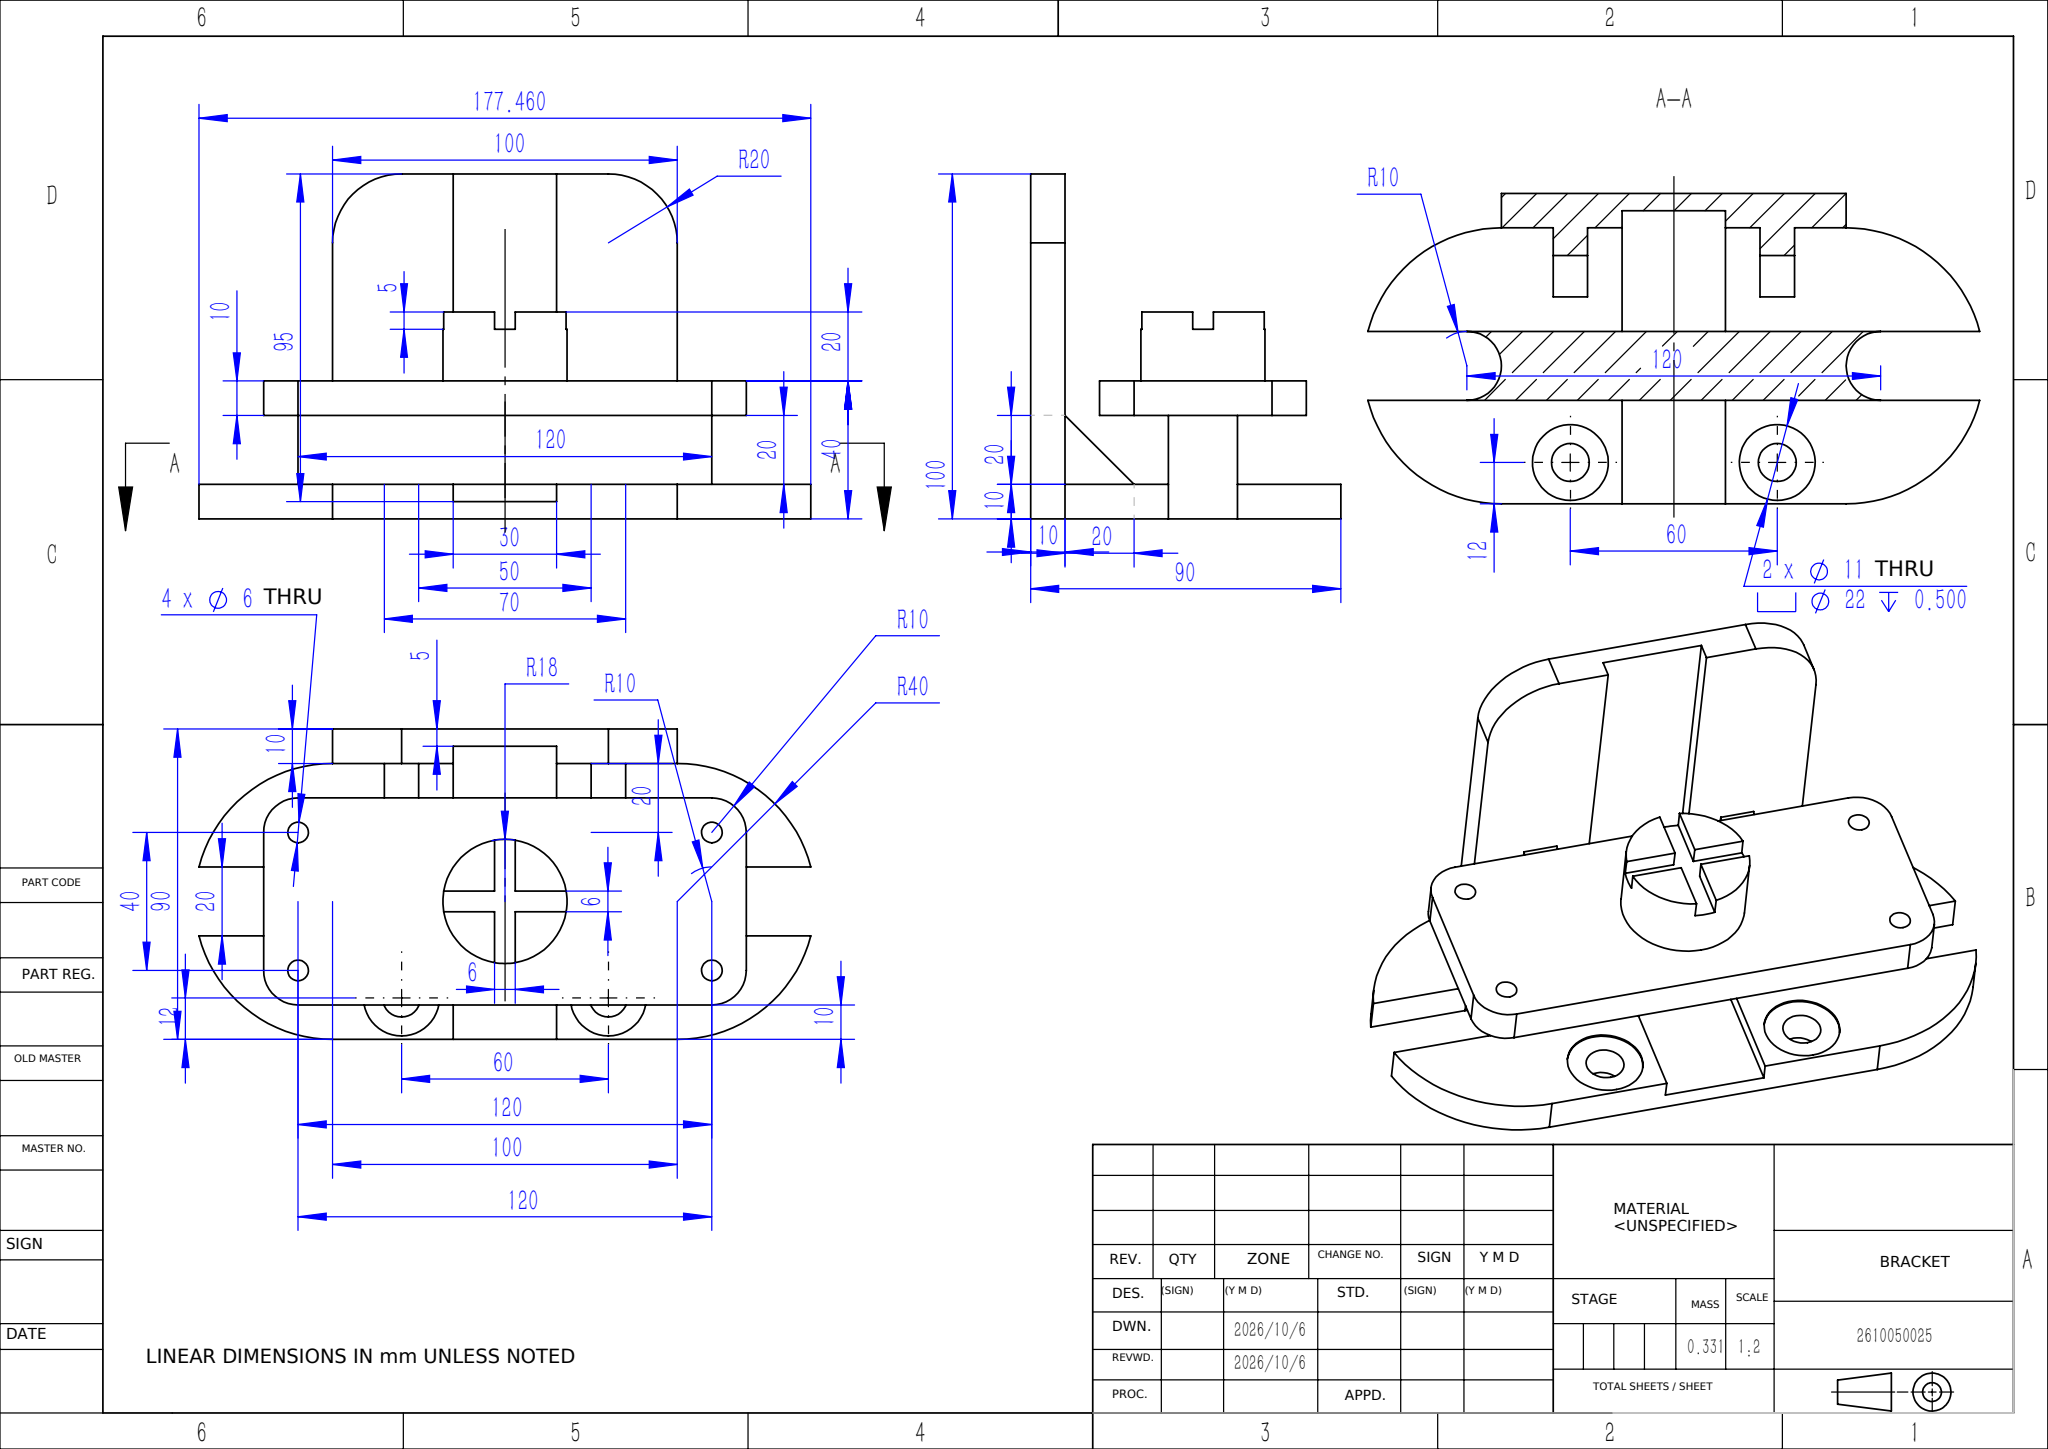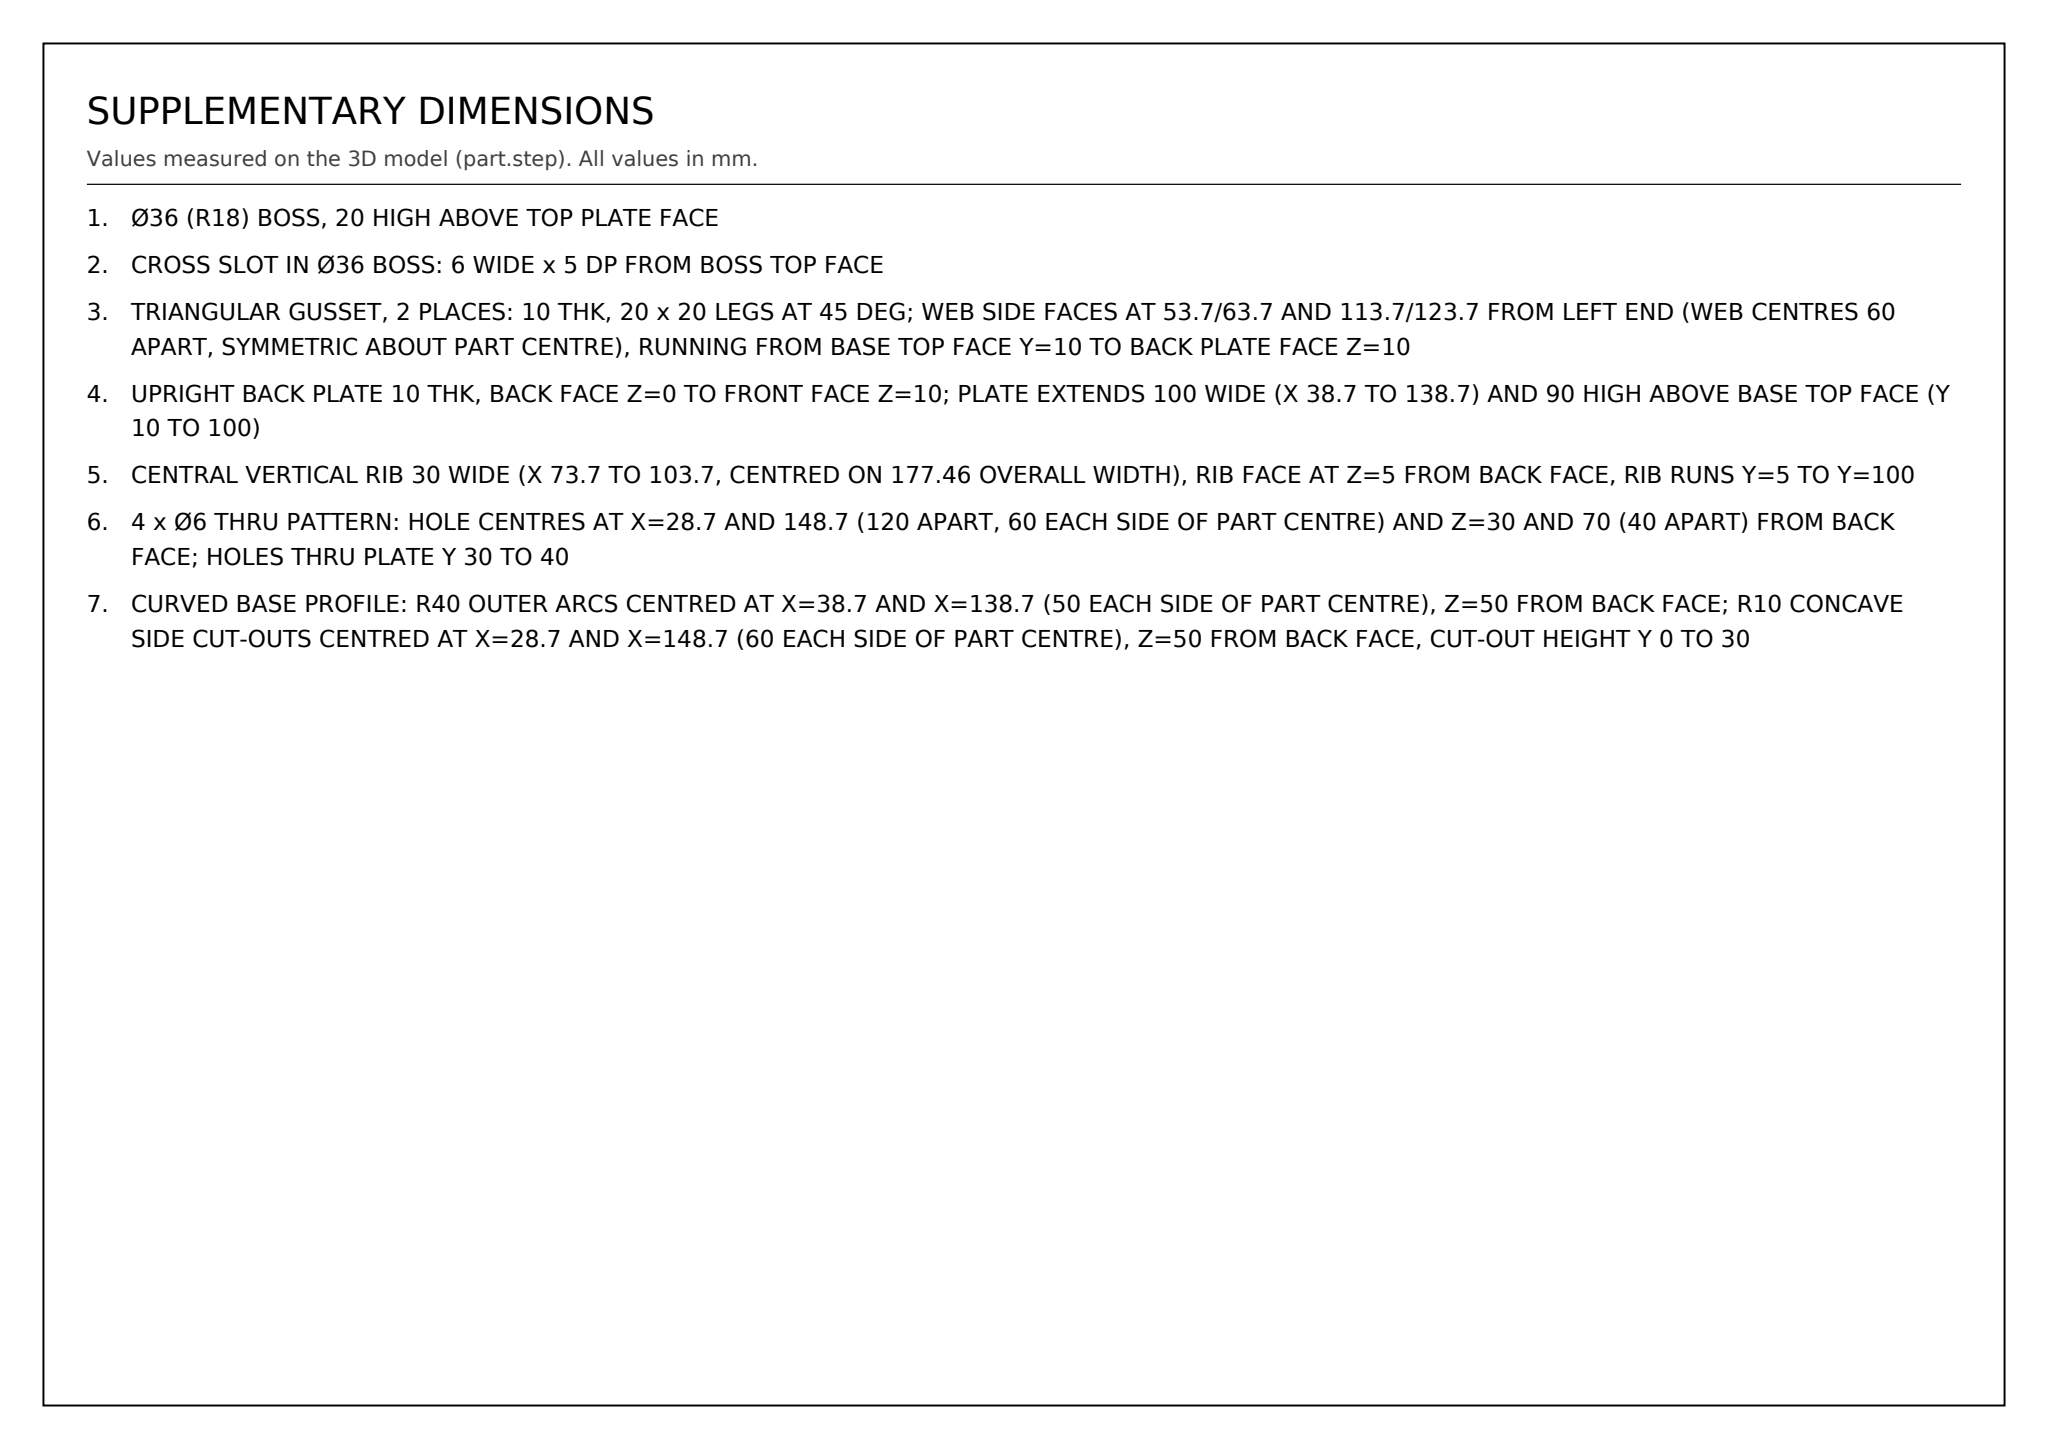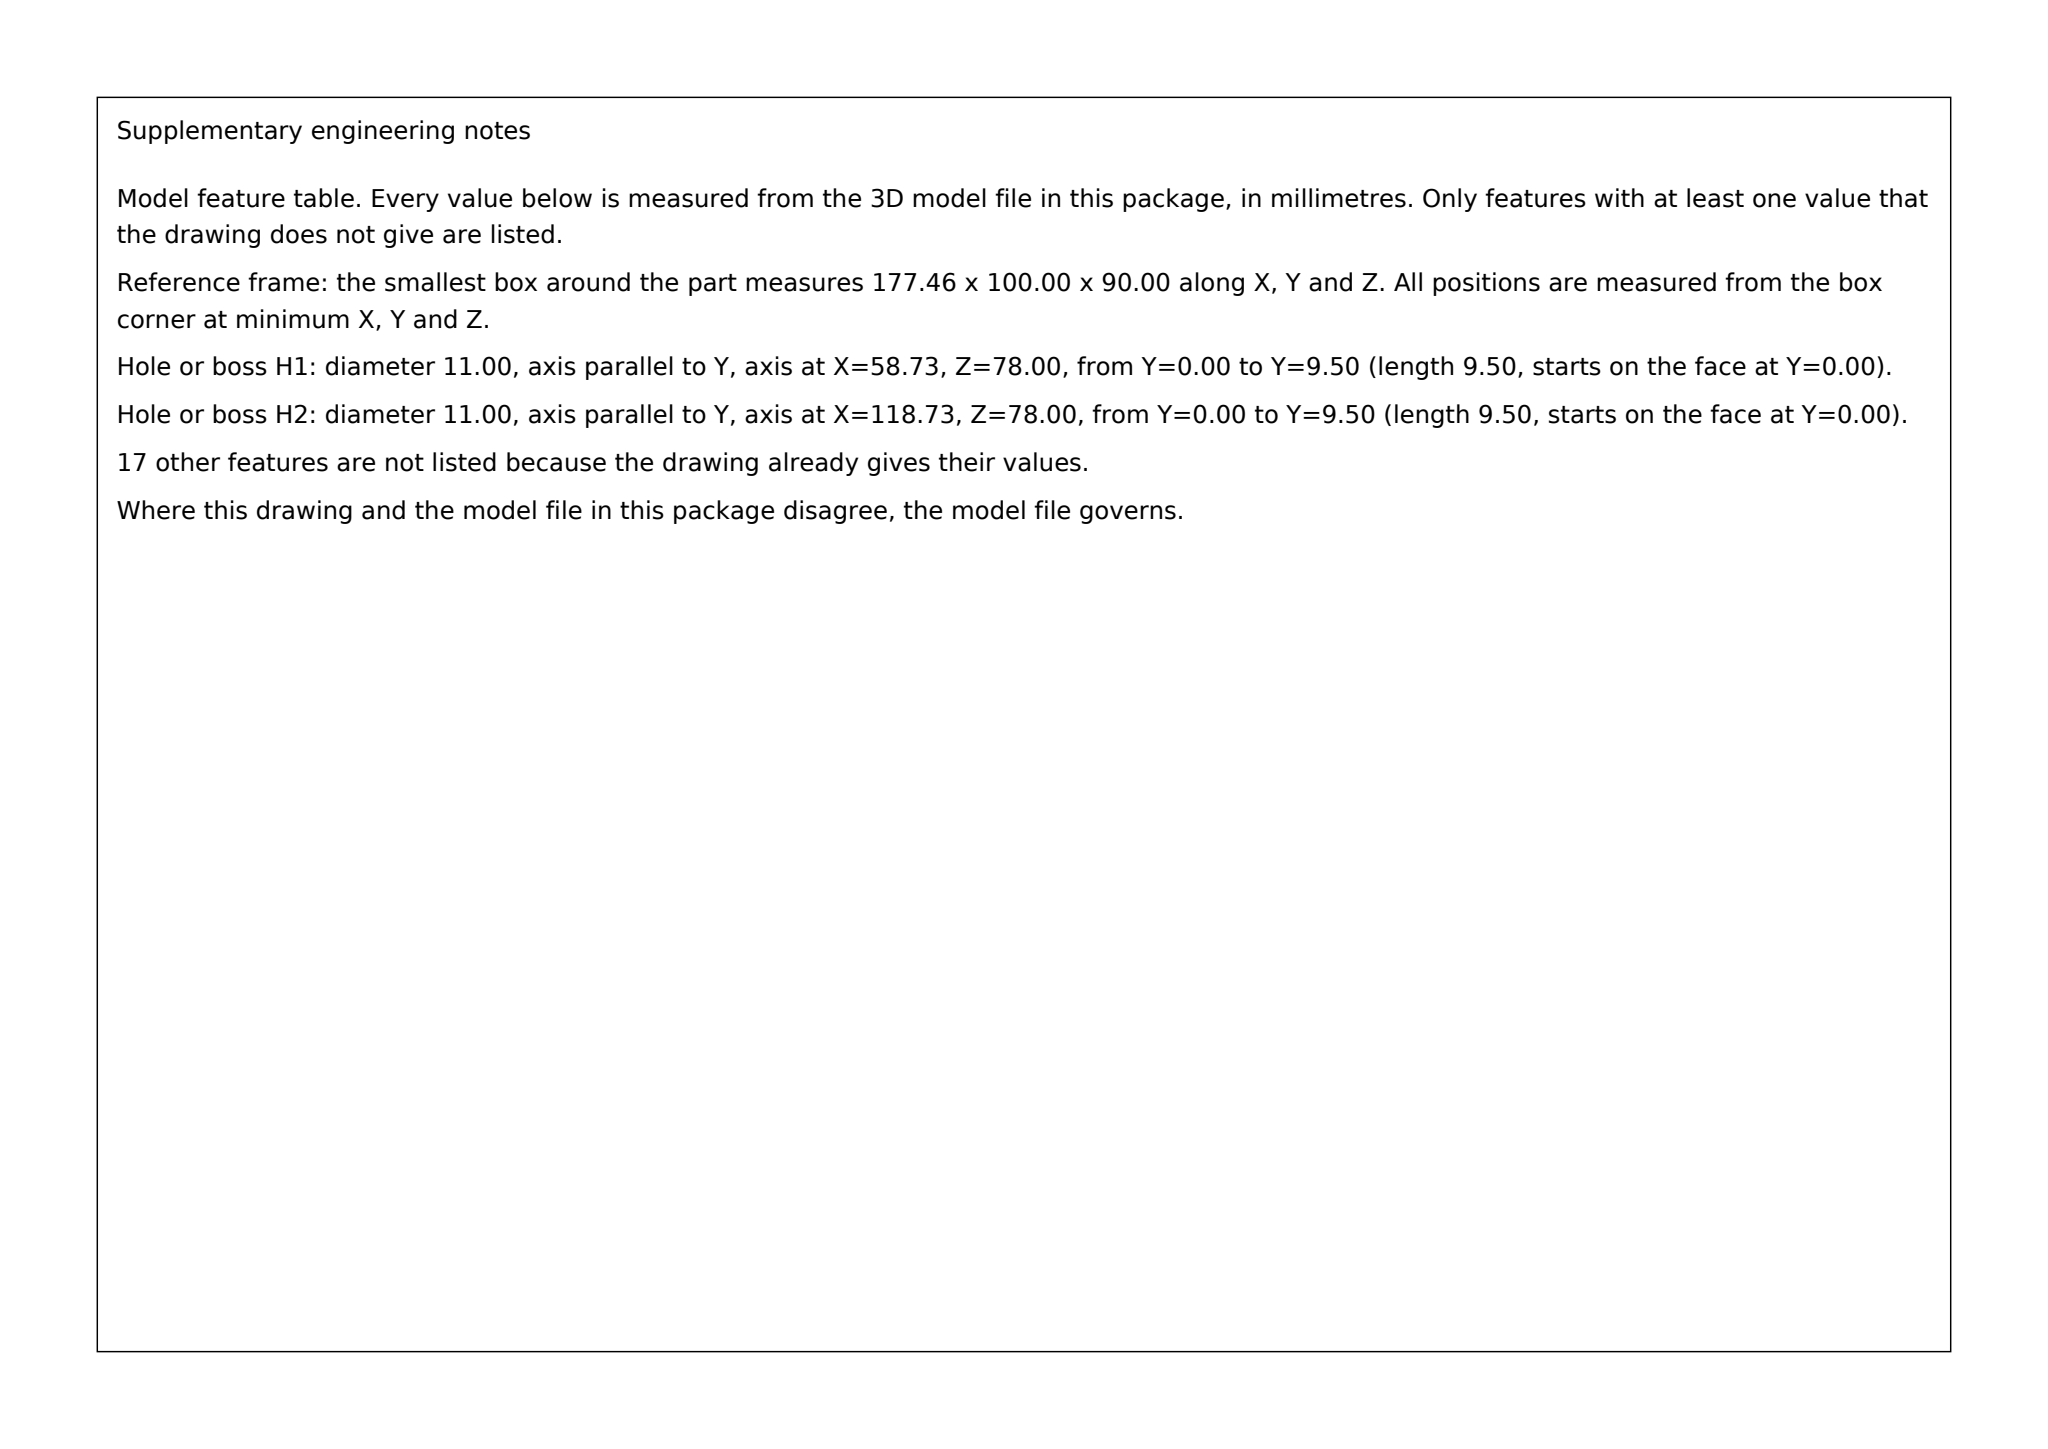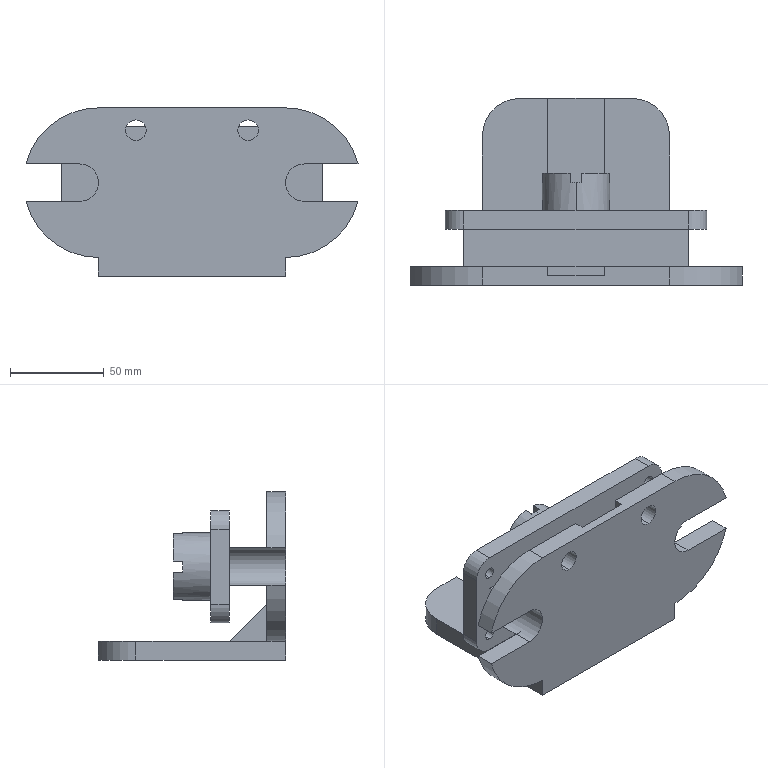Part | SolidWorks | mm | 1 solid | 80 faces | box 177.46 x 100 x 90 mm | volume 331255 mm3 | plane 50 | cylinder 30 | commonest cylinder face diameters 6 x8 20 x6 22 x4 11 x4 80 x4 36 x2 40 x2
Drawing notes:
Ø36 (R18) BOSS, 20 HIGH ABOVE TOP PLATE FACE | from the solid: Cylinder [36,y,(88.73,-,50.0),len 20]; plate top face y=40.0 to boss top y=60.0
CROSS SLOT IN Ø36 BOSS: 6 WIDE x 5 DP FROM BOSS TOP FACE | from the solid: Slot faces x=85.73/91.73 and z=47.0/53.0 (6 wide); boss top y=60.0, slot floor y=55.0 -> 5 deep
TRIANGULAR GUSSET, 2 PLACES: 10 THK, 20 x 20 LEGS AT 45 DEG; WEB SIDE FACES AT 53.7/63.7 AND 113.7/123.7 FROM LEFT END (WEB CENTRES 60 APART, SYMMETRIC ABOUT PART CENTRE), RUNNING FROM BASE TOP FACE Y=10 TO BACK PLATE FACE Z=10 | from the solid: inclined_planes angle_to_xyz [90,45,45], bbox_from [53.7,10,10] and [113.7,10,10], size [10,20,20]; x-planes 53.7/63.7/113.7/123.7 extent y[10,30] z[10,30] area 200
UPRIGHT BACK PLATE 10 THK, BACK FACE Z=0 TO FRONT FACE Z=10; PLATE EXTENDS 100 WIDE (X 38.7 TO 138.7) AND 90 HIGH ABOVE BASE TOP FACE (Y 10 TO 100) | from the solid: z-plane 0.0 extent x[38.7,138.7] y[0,100]; z-planes 10.0 extent x[38.7,73.7] and x[103.7,138.7], y[10,100]
CENTRAL VERTICAL RIB 30 WIDE (X 73.7 TO 103.7, CENTRED ON 177.46 OVERALL WIDTH), RIB FACE AT Z=5 FROM BACK FACE, RIB RUNS Y=5 TO Y=100 | from the solid: x-planes 73.7 and 103.7 extent y[5,100] z[5,90] area 875; z-plane 5.0 extent x[73.7,103.7] y[5,90] area 2850; y-plane 5.0 extent x[73.7,103.7] z[5,90] area 2550
4 x Ø6 THRU PATTERN: HOLE CENTRES AT X=28.7 AND 148.7 (120 APART, 60 EACH SIDE OF PART CENTRE) AND Z=30 AND 70 (40 APART) FROM BACK FACE; HOLES THRU PLATE Y 30 TO 40 | from the solid: cylinders hole/bore dia 6.0 axis y at [148.7,-,30], [148.7,-,70], [28.7,-,30], [28.7,-,70], from y 30.0 to 40.0
CURVED BASE PROFILE: R40 OUTER ARCS CENTRED AT X=38.7 AND X=138.7 (50 EACH SIDE OF PART CENTRE), Z=50 FROM BACK FACE; R10 CONCAVE SIDE CUT-OUTS CENTRED AT X=28.7 AND X=148.7 (60 EACH SIDE OF PART CENTRE), Z=50 FROM BACK FACE, CUT-OUT HEIGHT Y 0 TO 30 | from the solid: cylinders convex dia 80.0 axis y at [138.7,-,50] and [38.7,-,50] y 0 to 10 arc 151 deg; concave dia 20.0 axis y at [148.7,-,50] and [28.7,-,50] y 0 to 30 arc 180 deg
build123d program:
from build123d import *

# Parameters (mm, degrees)
BOSS_EXTRUDE1_DEPTH                                  = 10
SKETCH3_W                                            = 100
SKETCH3_H                                            = 10
BOSS_EXTRUDE2_DEPTH                                  = 100
FILLET1_R                                            = 20
CUT_EXTRUDE1_DEPTH                                   = 143.734
CUT_EXTRUDE1_DEPTH_BACK                              = 95
SKETCH4_W                                            = 30
SKETCH4_H                                            = 85
SKETCH5_W                                            = 10
SKETCH5_H                                            = 20
BOSS_EXTRUDE3_DEPTH                                  = 20
CUT_EXTRUDE2_DEPTH                                   = 20
CYLINDRICAL_COUNTERSUNK_HOLE_FOR_M10_HEX_D           = 11
CYLINDRICAL_COUNTERSUNK_HOLE_FOR_M10_HEX_CBORE_D     = 22
CYLINDRICAL_COUNTERSUNK_HOLE_FOR_M10_HEX_CBORE_DEPTH = 0.5
BOSS_EXTRUDE4_DEPTH                                  = 20
SKETCH11_W                                           = 140
SKETCH11_H                                           = 60
BOSS_EXTRUDE5_DEPTH                                  = 10
SKETCH12_R                                           = 18
BOSS_EXTRUDE6_DEPTH                                  = 20
CUT_EXTRUDE3_DEPTH                                   = 5
FILLET2_R                                            = 10
F_6_0MM_DOWEL_PIN_HOLE1_D                            = 6
F_6_0MM_DOWEL_PIN_HOLE1_DEPTH                        = 10


with BuildPart() as part:
    # Sketch1 → Boss-Extrude1 (new body)
    with BuildSketch(Plane(origin=(0, 0, 0), x_dir=(1, 0, 0), z_dir=(0, 1, 0))):
        with BuildLine():
            Line((-50, 40), (50, 40))
            ThreePointArc((50, 40), (74.495, 31.623), (88.73, 10))
            Line((88.73, 10), (60, 10))
            ThreePointArc((60, 10), (50, 0), (60, -10))
            Line((60, -10), (88.73, -10))
            ThreePointArc((88.73, -10), (74.495, -31.623), (50, -40))
            Line((50, -40), (-50, -40))
            ThreePointArc((-50, -40), (-74.495, -31.623), (-88.73, -10))
            Line((-88.73, -10), (-60, -10))
            ThreePointArc((-60, -10), (-50, 0), (-60, 10))
            Line((-60, 10), (-88.73, 10))
            ThreePointArc((-88.73, 10), (-74.495, 31.623), (-50, 40))
        make_face()
    extrude(amount=BOSS_EXTRUDE1_DEPTH)

    # Sketch3 → Boss-Extrude2 (add)
    with BuildSketch(Plane.XZ):
        with Locations((0, -45)):
            Rectangle(SKETCH3_W, SKETCH3_H)
    extrude(amount=-BOSS_EXTRUDE2_DEPTH)

    # Fillet1
    fillet1_edges = [part.edges().sort_by_distance(p)[0] for p in [
        (-50, 100, -45),
        (50, 100, -45),
    ]]
    fillet(fillet1_edges, radius=FILLET1_R)

    # Sketch4 → Cut-Extrude1 (cut, two sides: drawn at the far end of the back side and taken through both)
    with BuildSketch(Plane(origin=(0, 100, 0), x_dir=(1, 0, 0), z_dir=(0, 1, 0)).offset(-CUT_EXTRUDE1_DEPTH_BACK)):
        with Locations((0, 2.5)):
            Rectangle(SKETCH4_W, SKETCH4_H)
    extrude(amount=CUT_EXTRUDE1_DEPTH + CUT_EXTRUDE1_DEPTH_BACK, mode=Mode.SUBTRACT)

    # Sketch5 → Boss-Extrude3 (add)
    with BuildSketch(Plane.XY.offset(-40)):
        with Locations((-30, 20)):
            Rectangle(SKETCH5_W, SKETCH5_H)
    boss_extrude3 = extrude(amount=BOSS_EXTRUDE3_DEPTH)

    # Sketch6 → Cut-Extrude2 (cut)
    with BuildSketch(Plane.ZY.offset(35)):
        Polygon((-40, 30), (-20, 10), (-20, 30), align=None)
    cut_extrude2 = extrude(amount=-CUT_EXTRUDE2_DEPTH, mode=Mode.SUBTRACT)

    # Mirror1: Boss-Extrude3, Cut-Extrude2 across plane
    add(boss_extrude3.mirror(Plane(origin=(0, 0, 0), x_dir=(0, 0, 1), z_dir=(1, 0, 0))))
    add(cut_extrude2.mirror(Plane(origin=(0, 0, 0), x_dir=(0, 0, 1), z_dir=(1, 0, 0))), mode=Mode.SUBTRACT)

    # Cylindrical Countersunk Hole for M10 Hex (through all)
    with Locations(Plane(origin=(0, 10, 0), x_dir=(1, 0, 0), z_dir=(0, 1, 0))):
        with Locations((-30, -28), (30, -28)):
            CounterBoreHole(CYLINDRICAL_COUNTERSUNK_HOLE_FOR_M10_HEX_D / 2, CYLINDRICAL_COUNTERSUNK_HOLE_FOR_M10_HEX_CBORE_D / 2, CYLINDRICAL_COUNTERSUNK_HOLE_FOR_M10_HEX_CBORE_DEPTH)

    # Sketch10 → Boss-Extrude4 (add)
    with BuildSketch(Plane(origin=(0, 10, 0), x_dir=(1, 0, 0), z_dir=(0, 1, 0))):
        with BuildLine():
            Line((-60, 10), (60, 10))
            ThreePointArc((60, 10), (50, 0), (60, -10))
            Line((60, -10), (-60, -10))
            ThreePointArc((-60, -10), (-50, 0), (-60, 10))
        make_face()
    extrude(amount=BOSS_EXTRUDE4_DEPTH)

    # Sketch11 → Boss-Extrude5 (add)
    with BuildSketch(Plane(origin=(0, 30, 0), x_dir=(1, 0, 0), z_dir=(0, 1, 0))):
        Rectangle(SKETCH11_W, SKETCH11_H)
    extrude(amount=BOSS_EXTRUDE5_DEPTH)

    # Sketch12 → Boss-Extrude6 (add)
    with BuildSketch(Plane(origin=(0, 40, 0), x_dir=(1, 0, 0), z_dir=(0, 1, 0))):
        with Locations(Location((0, 0, 0), (0, 0, 270))):
            Circle(SKETCH12_R)
    extrude(amount=BOSS_EXTRUDE6_DEPTH)

    # Sketch13 → Cut-Extrude3 (cut)
    with BuildSketch(Plane(origin=(0, 60, 0), x_dir=(1, 0, 0), z_dir=(0, 1, 0))):
        Polygon((3, 3), (31.243, 3), (31.243, -3), (3, -3), (3, -24.197), (-3, -24.197), (-3, -3), (-31.243, -3), (-31.243, 3), (-3, 3), (-3, 24.197), (3, 24.197), align=None)
    extrude(amount=-CUT_EXTRUDE3_DEPTH, mode=Mode.SUBTRACT)

    # Fillet2
    fillet2_edges = [part.edges().sort_by_distance(p)[0] for p in [
        (70, 35, 30),
        (70, 35, -30),
        (-70, 35, -30),
        (-70, 35, 30),
    ]]
    fillet(fillet2_edges, radius=FILLET2_R)

    # 6.0mm Dowel Pin Hole1
    with Locations(Plane(origin=(0, 40, 0), x_dir=(1, 0, 0), z_dir=(0, 1, 0))):
        with Locations((-60, 20), (-60, -20), (60, -20), (60, 20)):
            Hole(F_6_0MM_DOWEL_PIN_HOLE1_D / 2, depth=F_6_0MM_DOWEL_PIN_HOLE1_DEPTH)


solid = part.part